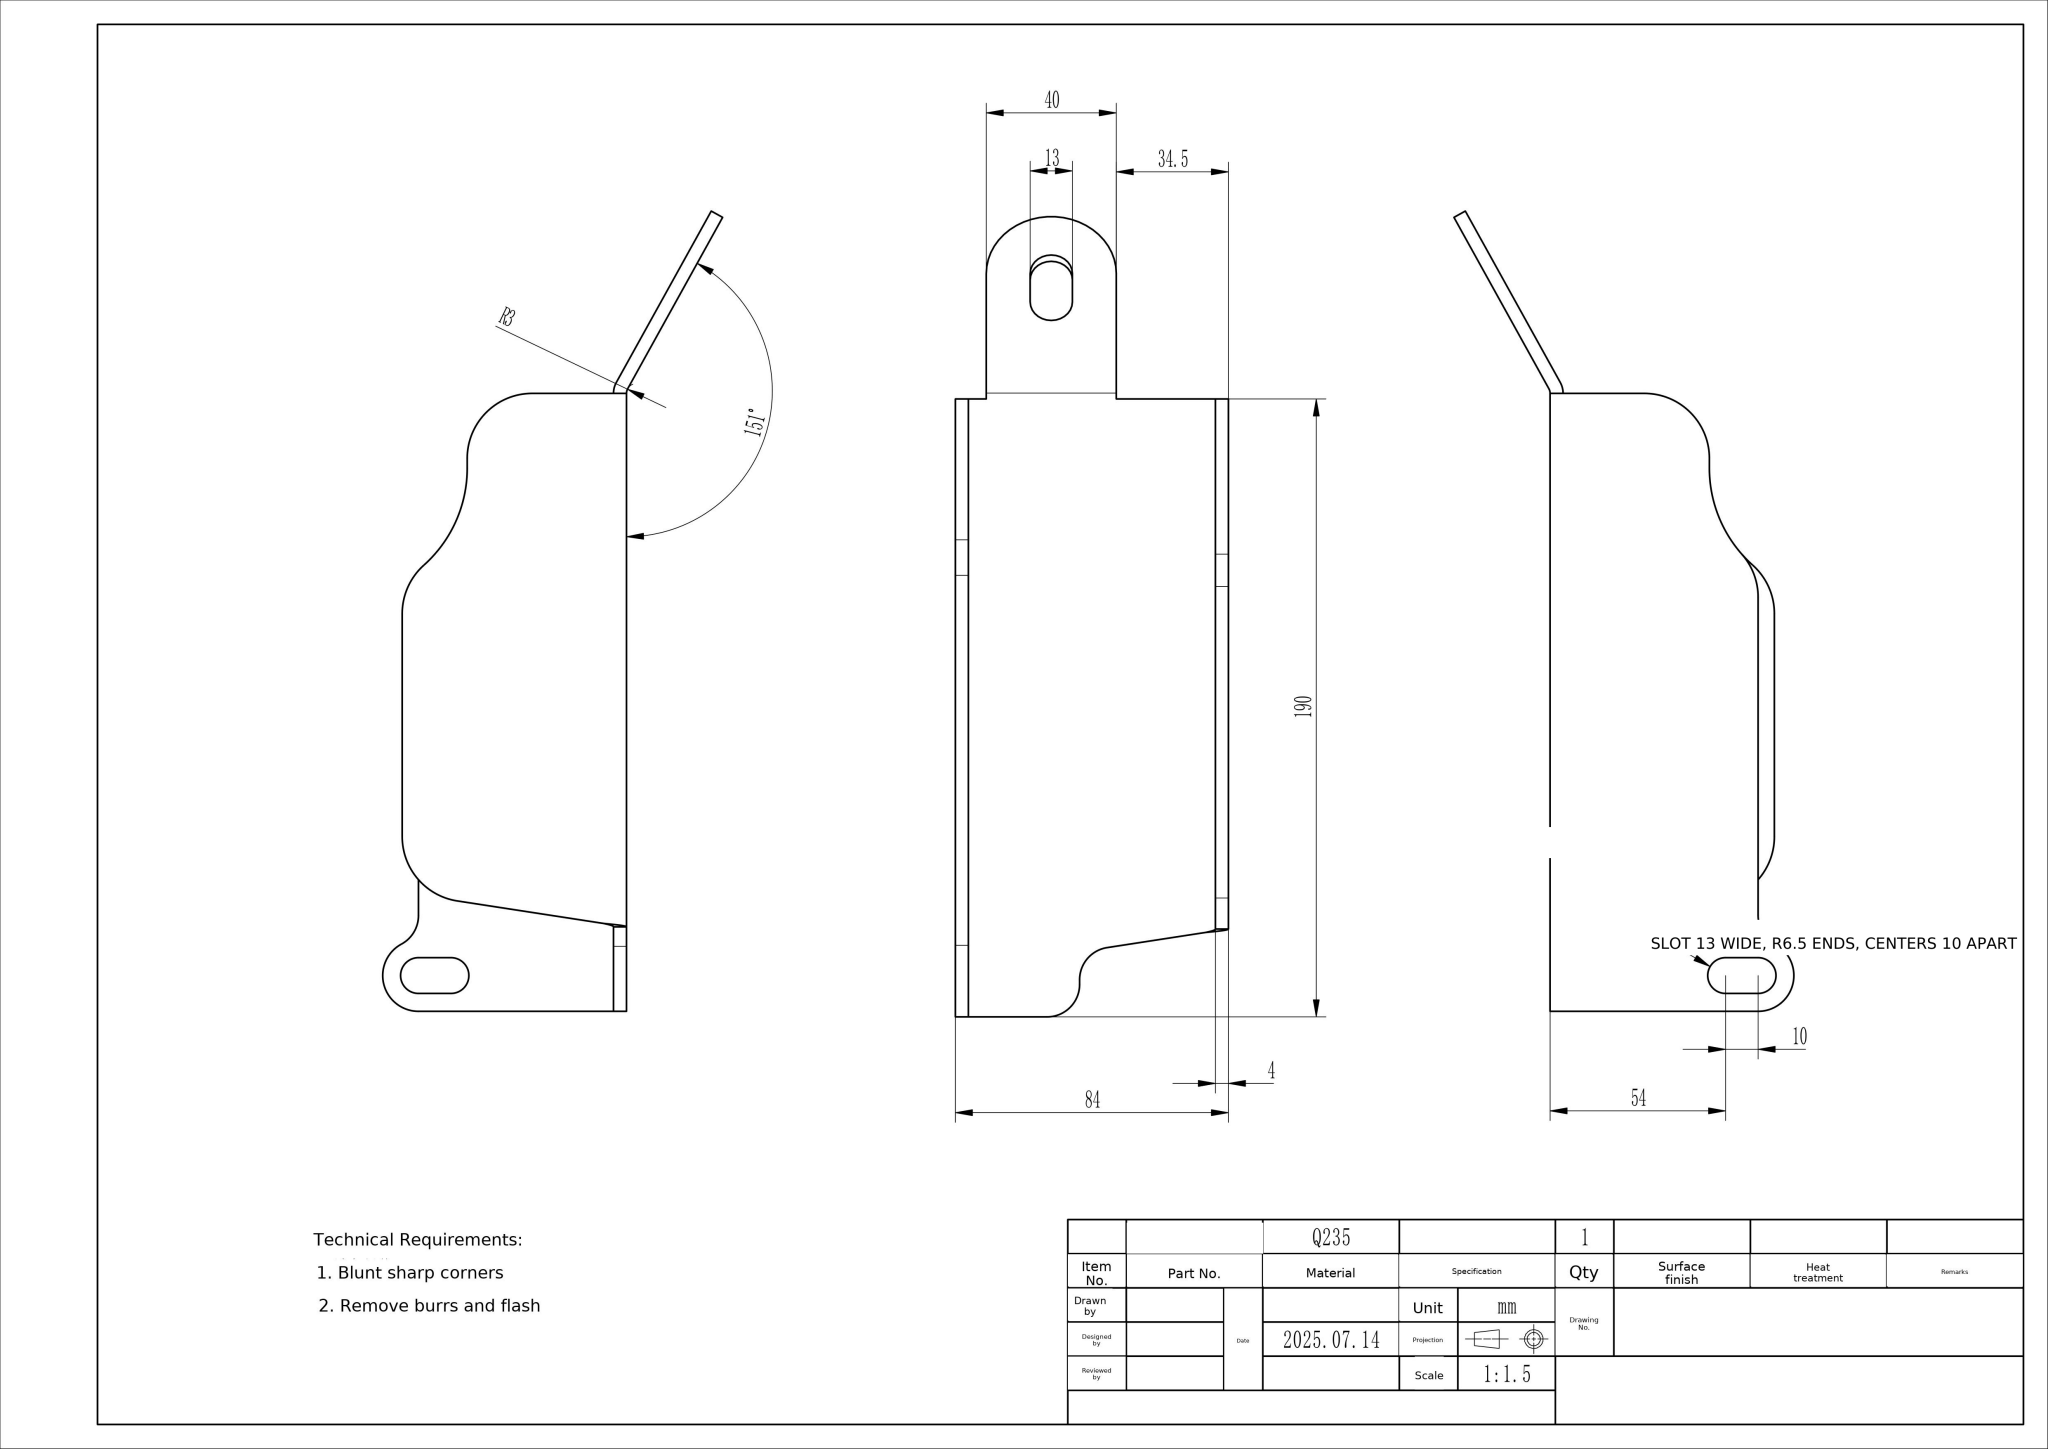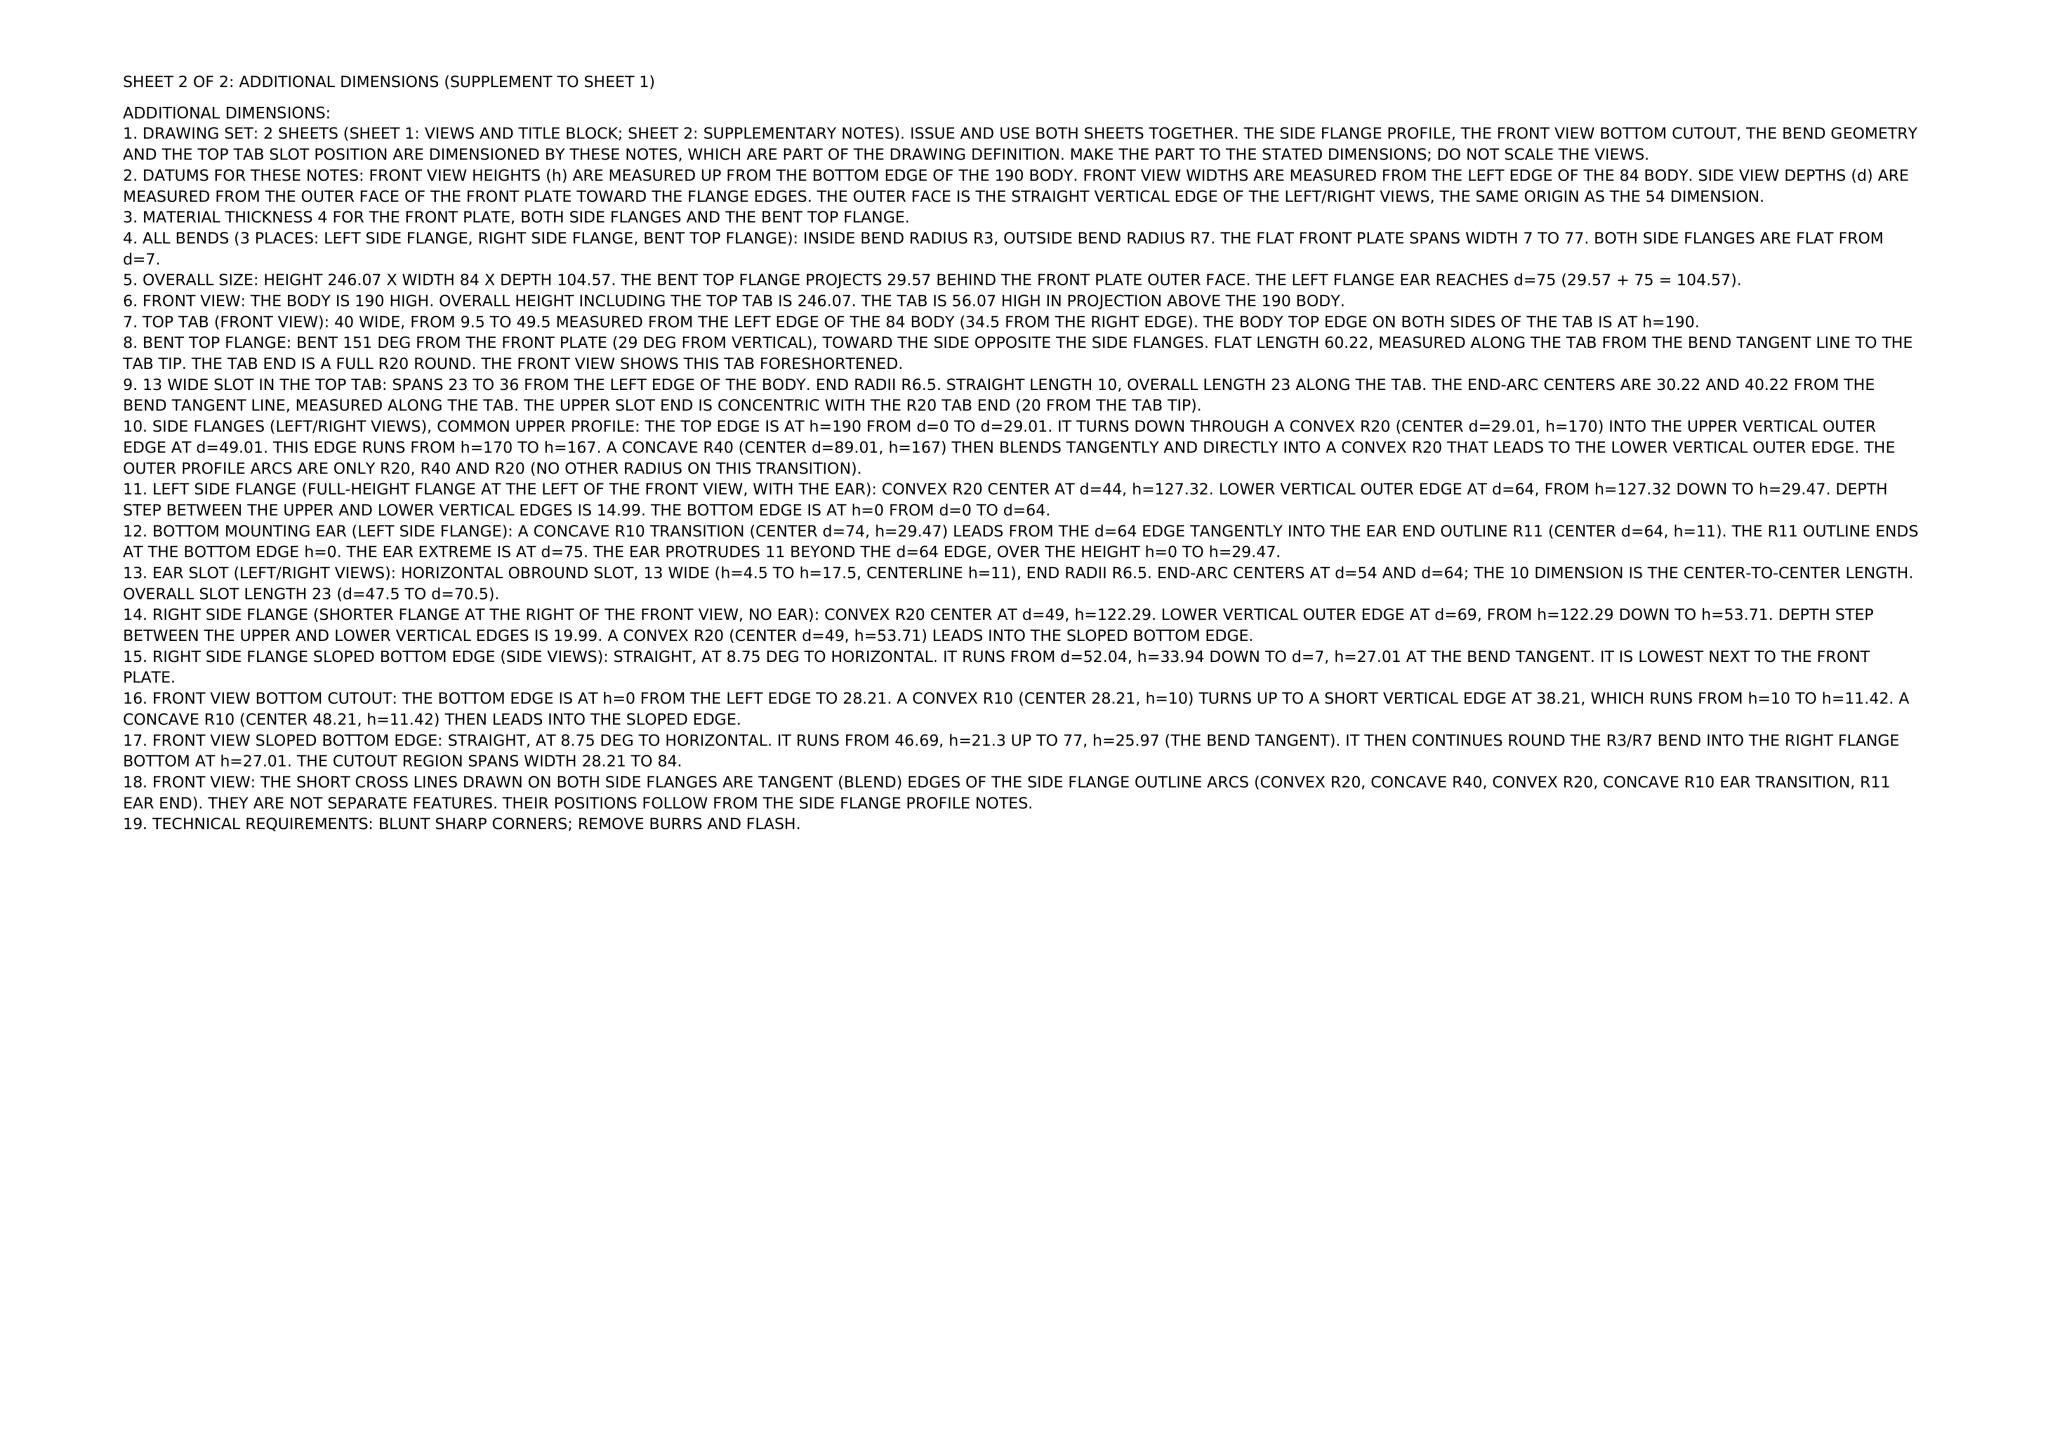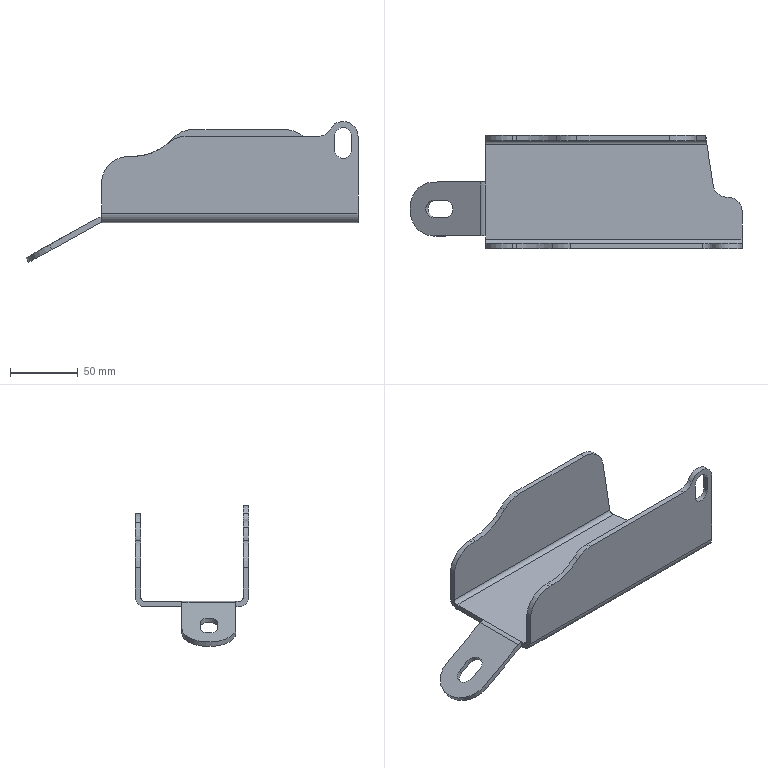Part | NX | mm | 1 solid | 47 faces | box 246.07 x 84 x 104.57 mm | volume 143821 mm3 | plane 24 | cylinder 22 | spline 1 | commonest cylinder face diameters 40 x6 13 x4 14 x3 6 x3 20 x3 80 x2 22 x1